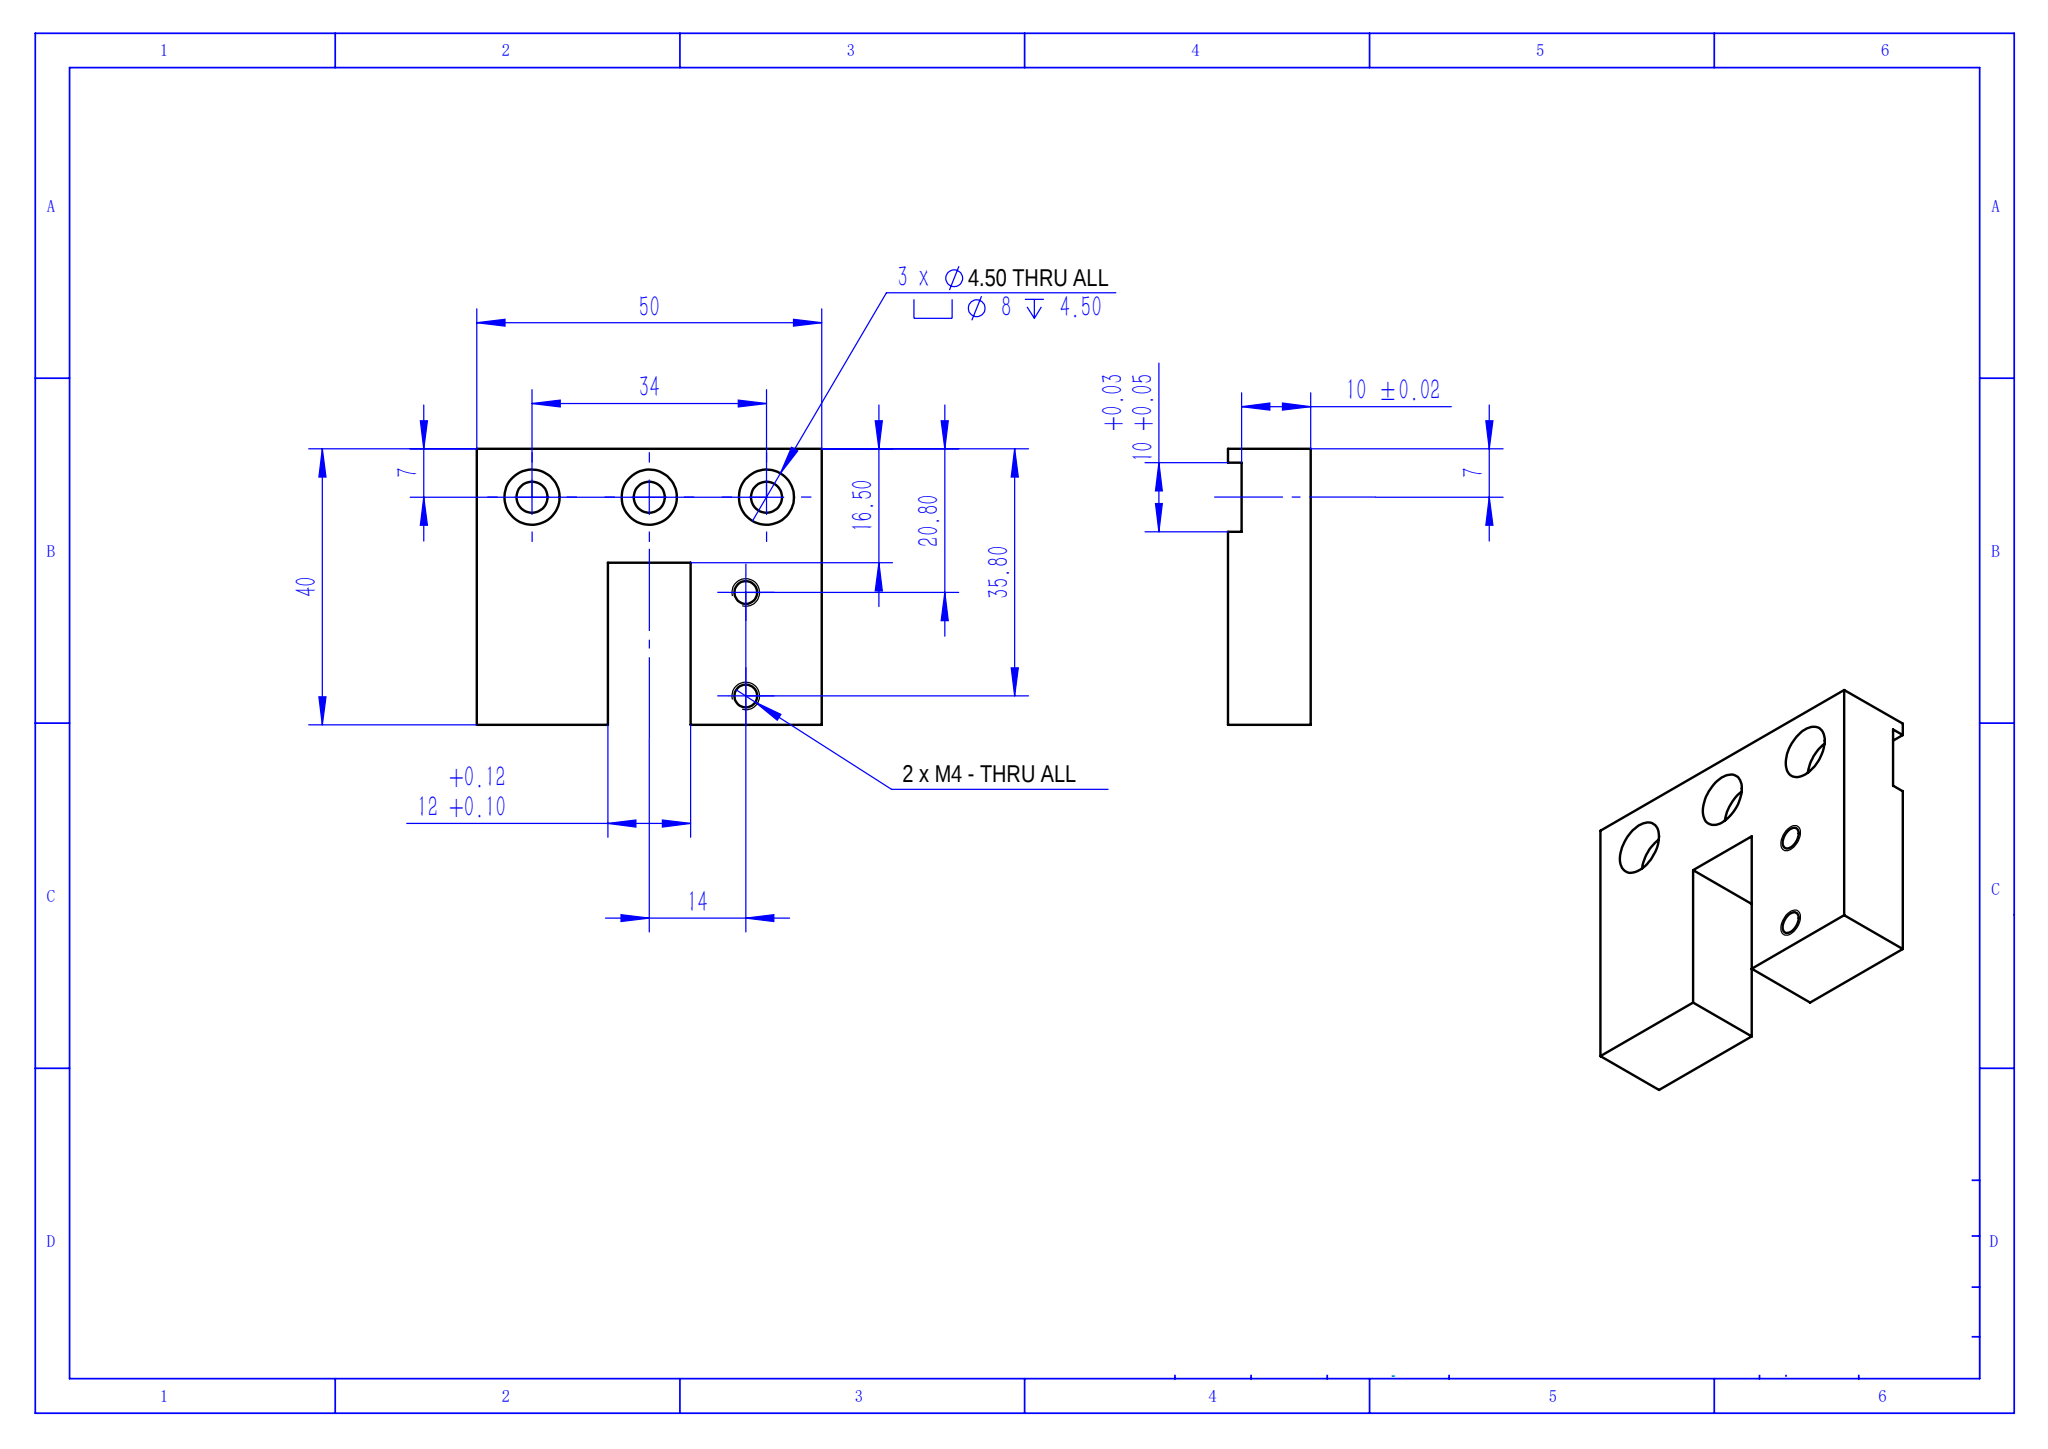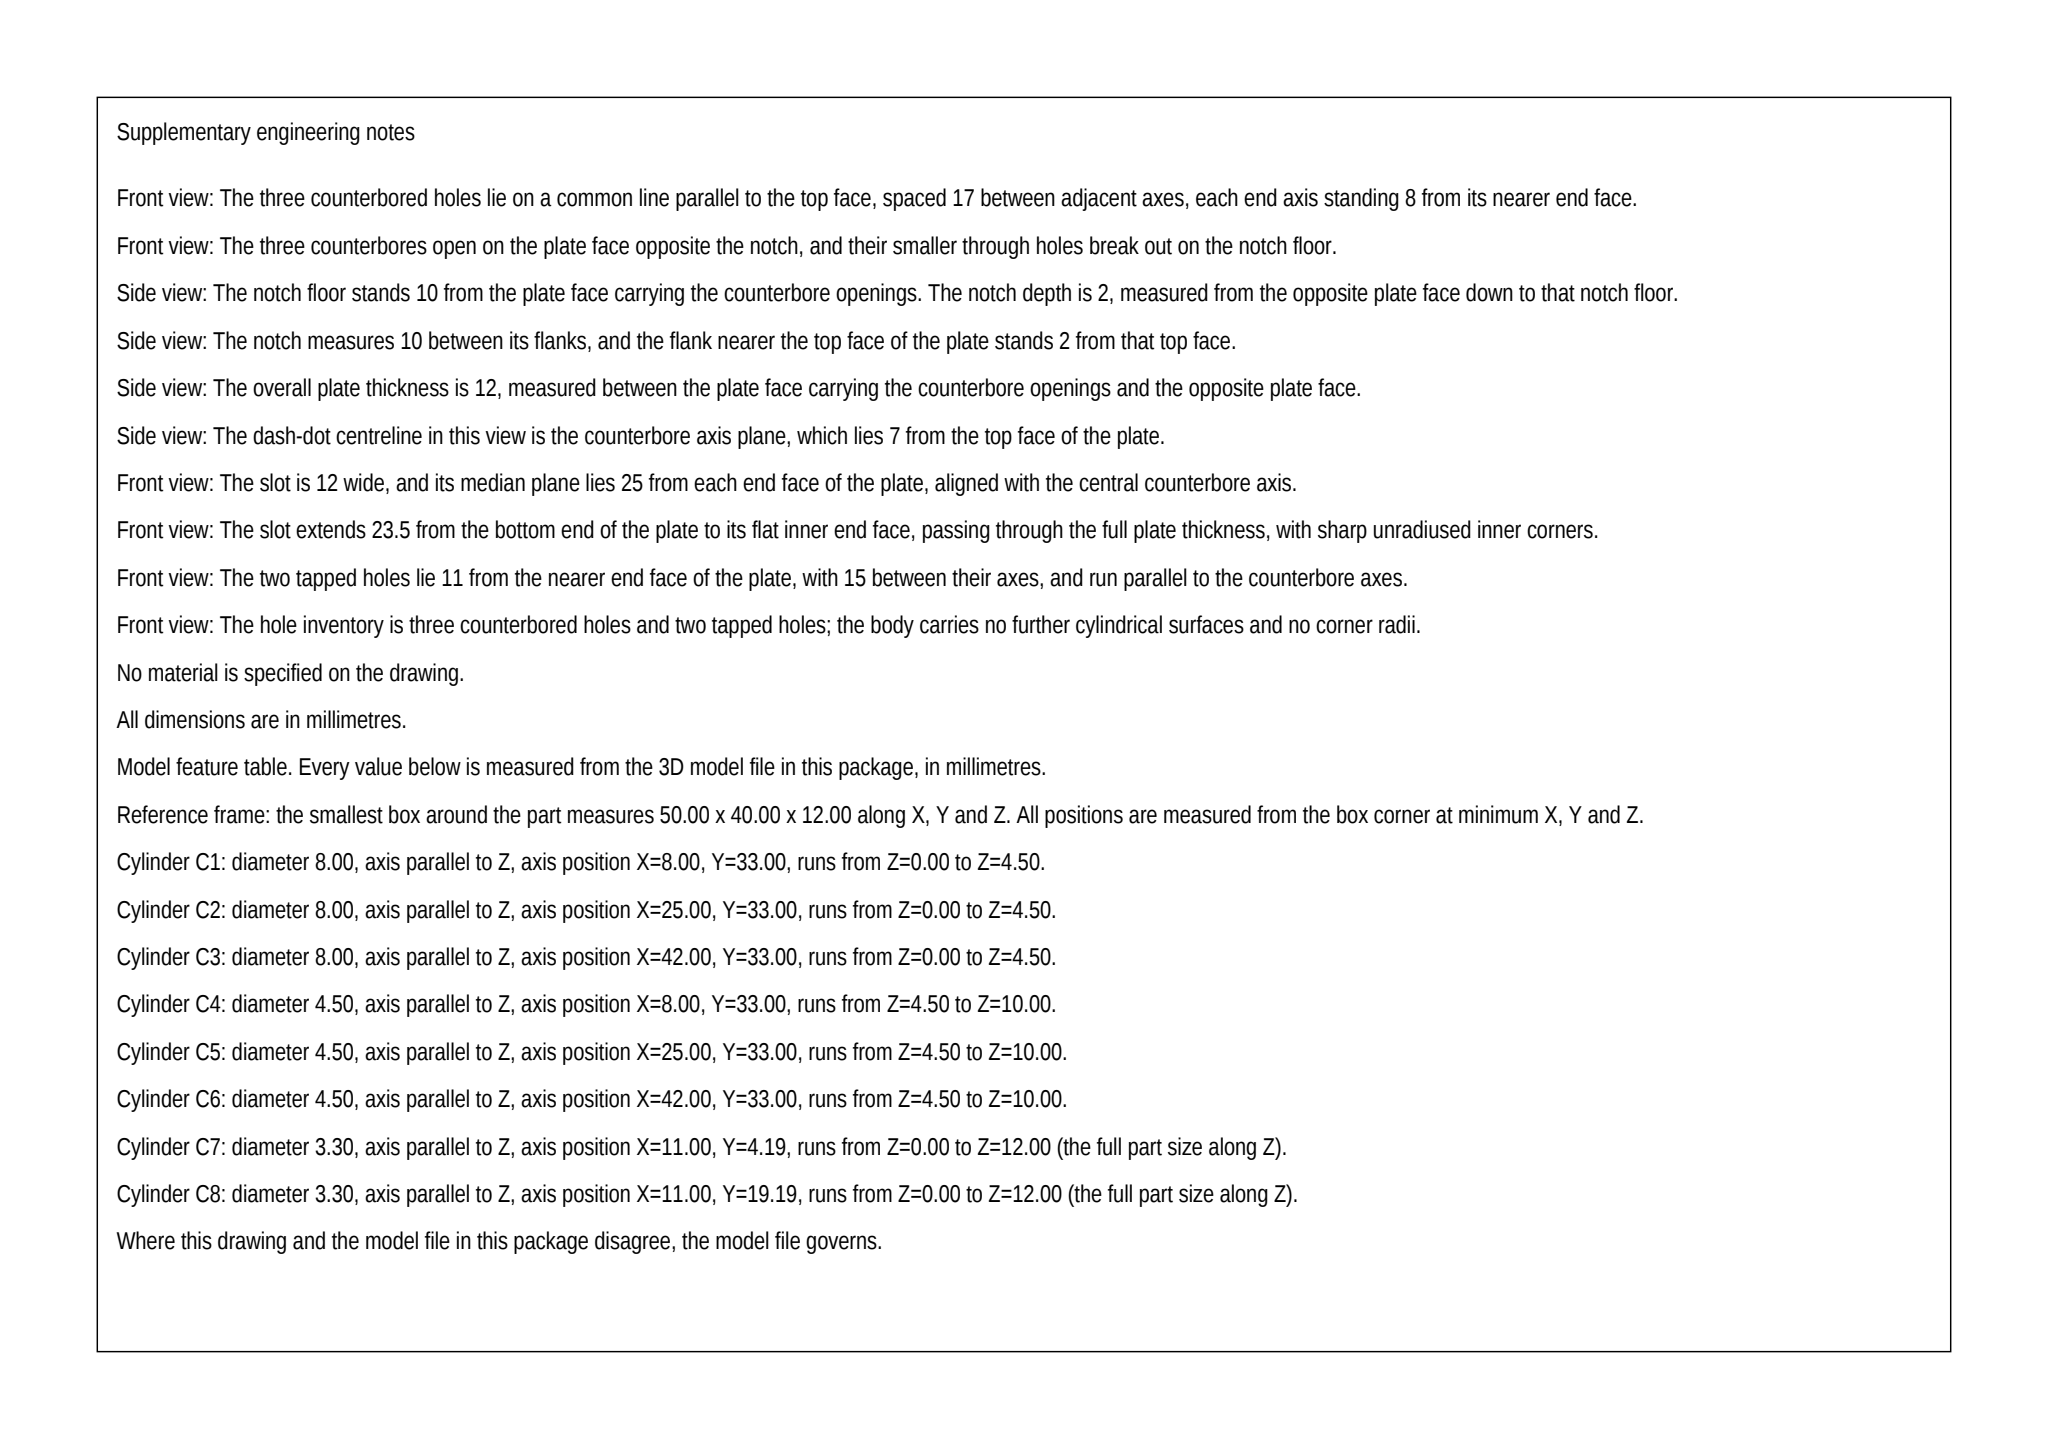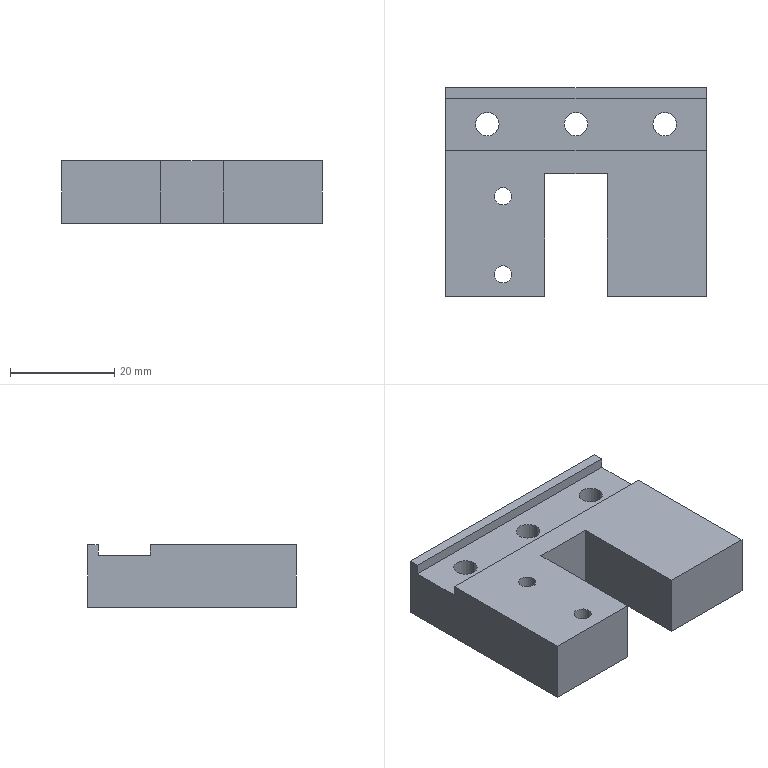Part | SolidWorks | mm | 1 solid | 33 faces | box 50 x 40 x 12 mm | volume 18470 mm3 | plane 17 | cylinder 16 | commonest cylinder face diameters 8 x6 4.5 x6 3.3 x4
Drawing notes:
SIDE VIEW: OVERALL THK 12; BACK FACE STEP 2 DEEP | from the solid: bbox z=12.0; z-planes at 10.0 and 12.0 give 2 step over 10 web
10 +0.03/+0.05 BACK RECESS: 2 DOWN FROM TOP FACE | from the solid: y-planes 28.0 and 38.0 (10 high) vs top face y=40.0 -> 2 offset
build123d program:
from build123d import *

# Parameters (mm, degrees)
SKETCH1_W                                            = 50
SKETCH1_H                                            = 40
BOSS_EXTRUDE1_DEPTH                                  = 20
SKETCH2_W                                            = 50
SKETCH2_H                                            = 10
CUT_EXTRUDE1_DEPTH                                   = 2
SKETCH3_W                                            = 19
SKETCH3_H                                            = 40
CUT_EXTRUDE3_DEPTH                                   = 8
SKETCH6_W                                            = 8
SKETCH6_H                                            = 23.5
CUT_EXTRUDE5_DEPTH                                   = 42.964
SKETCH7_W                                            = 12
SKETCH7_H                                            = 47
CUT_EXTRUDE6_DEPTH                                   = 56.172
SKETCH8_W                                            = 12
SKETCH8_H                                            = 16.5
CUT_EXTRUDE7_DEPTH                                   = 8
M4_HEX_HEAD_BOLT_CYLINDRICAL_COUNTERSUNK_D           = 4.5
M4_HEX_HEAD_BOLT_CYLINDRICAL_COUNTERSUNK_CBORE_D     = 8
M4_HEX_HEAD_BOLT_CYLINDRICAL_COUNTERSUNK_CBORE_DEPTH = 4.5
M4_TAPPED_HOLE1_D                                    = 3.3


with BuildPart() as part:
    # Sketch1 → Boss-Extrude1 (new body)
    with BuildSketch(Plane.XY):
        with Locations((25, 0)):
            Rectangle(SKETCH1_W, SKETCH1_H)
    extrude(amount=BOSS_EXTRUDE1_DEPTH)

    # Sketch2 → Cut-Extrude1 (cut)
    with BuildSketch(Plane.XY.offset(20)):
        with Locations((25, 13)):
            Rectangle(SKETCH2_W, SKETCH2_H)
    extrude(amount=-CUT_EXTRUDE1_DEPTH, mode=Mode.SUBTRACT)

    # Sketch3 → Cut-Extrude3 (cut)
    with BuildSketch(Plane(origin=(0, 0, 0), x_dir=(-1, 0, 0), z_dir=(0, 0, -1))):
        with Locations((-9.5, 0)):
            Rectangle(SKETCH3_W, SKETCH3_H)
        with Locations((-40.5, 0)):
            Rectangle(SKETCH3_W, SKETCH3_H)
    extrude(amount=-CUT_EXTRUDE3_DEPTH, mode=Mode.SUBTRACT)

    # Sketch6 → Cut-Extrude5 (cut, through all)
    with BuildSketch(Plane.ZY.offset(-19)):
        with Locations((4, -8.25)):
            Rectangle(SKETCH6_W, SKETCH6_H)
    extrude(amount=-CUT_EXTRUDE5_DEPTH, mode=Mode.SUBTRACT)

    # Sketch7 → Cut-Extrude6 (cut, through all)
    with BuildSketch(Plane(origin=(0, 0, 8), x_dir=(-1, 0, 0), z_dir=(0, 0, -1))):
        with Locations((-25, -20)):
            Rectangle(SKETCH7_W, SKETCH7_H)
    extrude(amount=-CUT_EXTRUDE6_DEPTH, mode=Mode.SUBTRACT)

    # Sketch8 → Cut-Extrude7 (cut)
    with BuildSketch(Plane(origin=(0, 0, 0), x_dir=(-1, 0, 0), z_dir=(0, 0, -1))):
        with Locations((-25, 11.75)):
            Rectangle(SKETCH8_W, SKETCH8_H)
    extrude(amount=-CUT_EXTRUDE7_DEPTH, mode=Mode.SUBTRACT)

    # M4 Hex Head Bolt Cylindrical Countersunk (through all)
    with Locations(Plane(origin=(0, 0, 8), x_dir=(-1, 0, 0), z_dir=(0, 0, -1))):
        with Locations((-42, 13), (-8, 13), (-25, 13)):
            CounterBoreHole(M4_HEX_HEAD_BOLT_CYLINDRICAL_COUNTERSUNK_D / 2, M4_HEX_HEAD_BOLT_CYLINDRICAL_COUNTERSUNK_CBORE_D / 2, M4_HEX_HEAD_BOLT_CYLINDRICAL_COUNTERSUNK_CBORE_DEPTH)

    # M4 Tapped Hole1 (through all)
    with Locations(Plane(origin=(11, -0.81, 8), x_dir=(-1, 0, 0), z_dir=(0, 0, -1))):
        with Locations((0, 0), (0, -15)):
            Hole(M4_TAPPED_HOLE1_D / 2)


solid = part.part